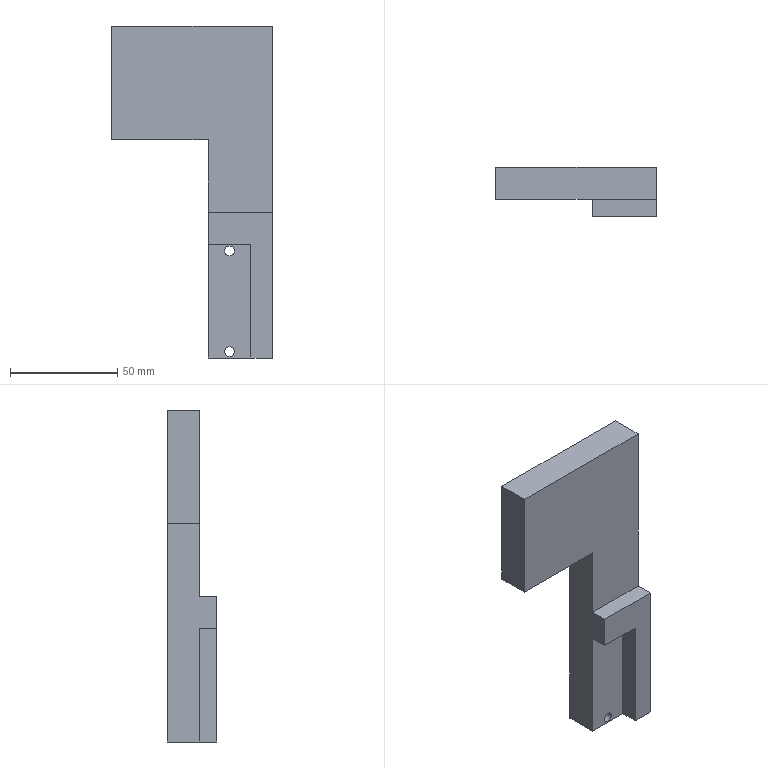Component | SolidWorks | TelescopicRodFixingBlock-1 | 1 solid | 24 faces | box 75 x 23 x 155 mm | volume 112588 mm3 | plane 15 | cylinder 9 | commonest cylinder face diameters 8 x5 4.5 x4
build123d program:
from build123d import *

# Parameters (mm, degrees)
BOSS_EXTRUDE1_DEPTH                             = 15
BOSS_EXTRUDE2_DEPTH                             = 8
M4_HEX_SOCKET_HEAD_CAP_SCREW_CBORE1_D           = 4.5
M4_HEX_SOCKET_HEAD_CAP_SCREW_CBORE1_CBORE_D     = 8
M4_HEX_SOCKET_HEAD_CAP_SCREW_CBORE1_CBORE_DEPTH = 4.6


with BuildPart() as part:
    # Sketch2 → Boss-Extrude1 (new body)
    with BuildSketch(Plane.XY):
        Polygon((10, 0.5), (-20, 0.5), (-20, 155.5), (55, 155.5), (55, 102.5), (10, 102.5), align=None)
    extrude(amount=BOSS_EXTRUDE1_DEPTH)

    # Sketch3 → Boss-Extrude2 (add)
    with BuildSketch(Plane(origin=(0, 0, 0), x_dir=(-1, 0, 0), z_dir=(0, 0, -1))):
        Polygon((20, 0.5), (10, 0.5), (10, 53.5), (-10, 53.5), (-10, 68.5), (20, 68.5), align=None)
    extrude(amount=BOSS_EXTRUDE2_DEPTH)

    # M4 Hex Socket Head Cap Screw CBORE1 (through all)
    with Locations(Plane.XY.offset(15)):
        with Locations((0, 50.5), (0, 3.5)):
            CounterBoreHole(M4_HEX_SOCKET_HEAD_CAP_SCREW_CBORE1_D / 2, M4_HEX_SOCKET_HEAD_CAP_SCREW_CBORE1_CBORE_D / 2, M4_HEX_SOCKET_HEAD_CAP_SCREW_CBORE1_CBORE_DEPTH)


solid = part.part

# Placed as in the assembly
solid = solid.moved(Location((-496.496, 273.496, 244.626), (-90, 0, 180)))
STEP:
#1=COLOUR_RGB('',0.7922,0.8196,0.9333);
#2=FILL_AREA_STYLE_COLOUR('',#1);
#3=FILL_AREA_STYLE('',(#2));
#4=SURFACE_STYLE_FILL_AREA(#3);
#5=SURFACE_SIDE_STYLE('',(#4));
#6=SURFACE_STYLE_USAGE(.BOTH.,#5);
#7=PRESENTATION_STYLE_ASSIGNMENT((#6));
#8=CARTESIAN_POINT('',(-19.39,11.177,11.619));
#9=VERTEX_POINT('',#8);
#10=CARTESIAN_POINT('',(-19.705,11.177,11.619));
#11=VERTEX_POINT('',#10);
#12=CARTESIAN_POINT('',(-19.547,11.177,11.619));
#13=DIRECTION('',(0.,1.,0.));
#14=DIRECTION('',(-1.,0.,0.));
#15=AXIS2_PLACEMENT_3D('',#12,#13,#14);
#16=CIRCLE('',#15,0.1575);
#17=EDGE_CURVE('',#9,#11,#16,.T.);
#18=ORIENTED_EDGE('',*,*,#17,.F.);
#19=CARTESIAN_POINT('',(-19.39,11.358,11.619));
#20=VERTEX_POINT('',#19);
#21=CARTESIAN_POINT('',(-19.39,11.358,11.619));
#22=DIRECTION('',(0.,1.,0.));
#23=VECTOR('',#22,39.37);
#24=LINE('',#21,#23);
#25=EDGE_CURVE('',#9,#20,#24,.T.);
#26=ORIENTED_EDGE('',*,*,#25,.T.);
#27=CARTESIAN_POINT('',(-19.705,11.358,11.619));
#28=VERTEX_POINT('',#27);
#29=CARTESIAN_POINT('',(-19.547,11.358,11.619));
#30=DIRECTION('',(0.,1.,0.));
#31=DIRECTION('',(-1.,0.,0.));
#32=AXIS2_PLACEMENT_3D('',#29,#30,#31);
#33=CIRCLE('',#32,0.1575);
#34=EDGE_CURVE('',#20,#28,#33,.T.);
#35=ORIENTED_EDGE('',*,*,#34,.T.);
#36=CARTESIAN_POINT('',(-19.705,11.358,11.619));
#37=DIRECTION('',(0.,1.,0.));
#38=VECTOR('',#37,39.37);
#39=LINE('',#36,#38);
#40=EDGE_CURVE('',#11,#28,#39,.T.);
#41=ORIENTED_EDGE('',*,*,#40,.F.);
#42=EDGE_LOOP('',(#18,#26,#35,#41));
#43=FACE_OUTER_BOUND('',#42,.T.);
#44=CARTESIAN_POINT('',(-19.547,11.358,11.619));
#45=DIRECTION('',(0.,1.,0.));
#46=DIRECTION('',(-1.,0.,0.));
#47=AXIS2_PLACEMENT_3D('',#44,#45,#46);
#48=CYLINDRICAL_SURFACE('',#47,0.1575);
#49=ADVANCED_FACE('',(#43),#48,.F.);
#50=CARTESIAN_POINT('',(-19.636,10.768,11.619));
#51=VERTEX_POINT('',#50);
#52=CARTESIAN_POINT('',(-19.459,10.768,11.619));
#53=VERTEX_POINT('',#52);
#54=CARTESIAN_POINT('',(-19.547,10.768,11.619));
#55=DIRECTION('',(-0.,-1.,-0.));
#56=DIRECTION('',(1.,0.,0.));
#57=AXIS2_PLACEMENT_3D('',#54,#55,#56);
#58=CIRCLE('',#57,0.08858);
#59=EDGE_CURVE('',#51,#53,#58,.T.);
#60=ORIENTED_EDGE('',*,*,#59,.T.);
#61=CARTESIAN_POINT('',(-19.459,11.177,11.619));
#62=VERTEX_POINT('',#61);
#63=CARTESIAN_POINT('',(-19.459,11.358,11.619));
#64=DIRECTION('',(0.,1.,0.));
#65=VECTOR('',#64,39.37);
#66=LINE('',#63,#65);
#67=EDGE_CURVE('',#53,#62,#66,.T.);
#68=ORIENTED_EDGE('',*,*,#67,.T.);
#69=CARTESIAN_POINT('',(-19.636,11.177,11.619));
#70=VERTEX_POINT('',#69);
#71=CARTESIAN_POINT('',(-19.547,11.177,11.619));
#72=DIRECTION('',(0.,1.,0.));
#73=DIRECTION('',(-1.,0.,0.));
#74=AXIS2_PLACEMENT_3D('',#71,#72,#73);
#75=CIRCLE('',#74,0.08858);
#76=EDGE_CURVE('',#62,#70,#75,.T.);
#77=ORIENTED_EDGE('',*,*,#76,.T.);
#78=CARTESIAN_POINT('',(-19.636,11.358,11.619));
#79=DIRECTION('',(0.,1.,0.));
#80=VECTOR('',#79,39.37);
#81=LINE('',#78,#80);
#82=EDGE_CURVE('',#51,#70,#81,.T.);
#83=ORIENTED_EDGE('',*,*,#82,.F.);
#84=EDGE_LOOP('',(#60,#68,#77,#83));
#85=FACE_OUTER_BOUND('',#84,.T.);
#86=CARTESIAN_POINT('',(-19.547,11.358,11.619));
#87=DIRECTION('',(0.,1.,0.));
#88=DIRECTION('',(-1.,0.,0.));
#89=AXIS2_PLACEMENT_3D('',#86,#87,#88);
#90=CYLINDRICAL_SURFACE('',#89,0.08858);
#91=ADVANCED_FACE('',(#85),#90,.F.);
#92=CARTESIAN_POINT('',(-19.636,10.768,9.769));
#93=VERTEX_POINT('',#92);
#94=CARTESIAN_POINT('',(-19.459,10.768,9.769));
#95=VERTEX_POINT('',#94);
#96=CARTESIAN_POINT('',(-19.547,10.768,9.769));
#97=DIRECTION('',(-0.,-1.,-0.));
#98=DIRECTION('',(1.,0.,0.));
#99=AXIS2_PLACEMENT_3D('',#96,#97,#98);
#100=CIRCLE('',#99,0.08858);
#101=EDGE_CURVE('',#93,#95,#100,.T.);
#102=ORIENTED_EDGE('',*,*,#101,.T.);
#103=CARTESIAN_POINT('',(-19.459,11.177,9.769));
#104=VERTEX_POINT('',#103);
#105=CARTESIAN_POINT('',(-19.459,11.358,9.769));
#106=DIRECTION('',(0.,1.,0.));
#107=VECTOR('',#106,39.37);
#108=LINE('',#105,#107);
#109=EDGE_CURVE('',#95,#104,#108,.T.);
#110=ORIENTED_EDGE('',*,*,#109,.T.);
#111=CARTESIAN_POINT('',(-19.636,11.177,9.769));
#112=VERTEX_POINT('',#111);
#113=CARTESIAN_POINT('',(-19.547,11.177,9.769));
#114=DIRECTION('',(0.,1.,0.));
#115=DIRECTION('',(-1.,0.,0.));
#116=AXIS2_PLACEMENT_3D('',#113,#114,#115);
#117=CIRCLE('',#116,0.08858);
#118=EDGE_CURVE('',#104,#112,#117,.T.);
#119=ORIENTED_EDGE('',*,*,#118,.T.);
#120=CARTESIAN_POINT('',(-19.636,11.358,9.769));
#121=DIRECTION('',(0.,1.,0.));
#122=VECTOR('',#121,39.37);
#123=LINE('',#120,#122);
#124=EDGE_CURVE('',#93,#112,#123,.T.);
#125=ORIENTED_EDGE('',*,*,#124,.F.);
#126=EDGE_LOOP('',(#102,#110,#119,#125));
#127=FACE_OUTER_BOUND('',#126,.T.);
#128=CARTESIAN_POINT('',(-19.547,11.358,9.769));
#129=DIRECTION('',(0.,1.,0.));
#130=DIRECTION('',(-1.,0.,0.));
#131=AXIS2_PLACEMENT_3D('',#128,#129,#130);
#132=CYLINDRICAL_SURFACE('',#131,0.08858);
#133=ADVANCED_FACE('',(#127),#132,.F.);
#134=CARTESIAN_POINT('',(-19.39,11.177,9.769));
#135=VERTEX_POINT('',#134);
#136=CARTESIAN_POINT('',(-19.443,11.177,9.651));
#137=VERTEX_POINT('',#136);
#138=CARTESIAN_POINT('',(-19.547,11.177,9.769));
#139=DIRECTION('',(0.,1.,0.));
#140=DIRECTION('',(-1.,0.,0.));
#141=AXIS2_PLACEMENT_3D('',#138,#139,#140);
#142=CIRCLE('',#141,0.1575);
#143=EDGE_CURVE('',#135,#137,#142,.T.);
#144=ORIENTED_EDGE('',*,*,#143,.F.);
#145=CARTESIAN_POINT('',(-19.39,11.358,9.769));
#146=VERTEX_POINT('',#145);
#147=CARTESIAN_POINT('',(-19.39,11.358,9.769));
#148=DIRECTION('',(0.,1.,0.));
#149=VECTOR('',#148,39.37);
#150=LINE('',#147,#149);
#151=EDGE_CURVE('',#135,#146,#150,.T.);
#152=ORIENTED_EDGE('',*,*,#151,.T.);
#153=CARTESIAN_POINT('',(-19.443,11.358,9.651));
#154=VERTEX_POINT('',#153);
#155=CARTESIAN_POINT('',(-19.547,11.358,9.769));
#156=DIRECTION('',(0.,1.,0.));
#157=DIRECTION('',(-1.,0.,0.));
#158=AXIS2_PLACEMENT_3D('',#155,#156,#157);
#159=CIRCLE('',#158,0.1575);
#160=EDGE_CURVE('',#146,#154,#159,.T.);
#161=ORIENTED_EDGE('',*,*,#160,.T.);
#162=CARTESIAN_POINT('',(-19.443,11.358,9.651));
#163=DIRECTION('',(0.,1.,0.));
#164=VECTOR('',#163,39.37);
#165=LINE('',#162,#164);
#166=EDGE_CURVE('',#137,#154,#165,.T.);
#167=ORIENTED_EDGE('',*,*,#166,.F.);
#168=EDGE_LOOP('',(#144,#152,#161,#167));
#169=FACE_OUTER_BOUND('',#168,.T.);
#170=CARTESIAN_POINT('',(-19.547,11.358,9.769));
#171=DIRECTION('',(0.,1.,0.));
#172=DIRECTION('',(-1.,0.,0.));
#173=AXIS2_PLACEMENT_3D('',#170,#171,#172);
#174=CYLINDRICAL_SURFACE('',#173,0.1575);
#175=ADVANCED_FACE('',(#169),#174,.F.);
#176=ORIENTED_EDGE('',*,*,#151,.F.);
#177=CARTESIAN_POINT('',(-19.705,11.177,9.769));
#178=VERTEX_POINT('',#177);
#179=CARTESIAN_POINT('',(-19.547,11.177,9.769));
#180=DIRECTION('',(0.,1.,0.));
#181=DIRECTION('',(-1.,0.,0.));
#182=AXIS2_PLACEMENT_3D('',#179,#180,#181);
#183=CIRCLE('',#182,0.1575);
#184=EDGE_CURVE('',#178,#135,#183,.T.);
#185=ORIENTED_EDGE('',*,*,#184,.F.);
#186=CARTESIAN_POINT('',(-19.705,11.358,9.769));
#187=VERTEX_POINT('',#186);
#188=CARTESIAN_POINT('',(-19.705,11.358,9.769));
#189=DIRECTION('',(0.,1.,0.));
#190=VECTOR('',#189,39.37);
#191=LINE('',#188,#190);
#192=EDGE_CURVE('',#178,#187,#191,.T.);
#193=ORIENTED_EDGE('',*,*,#192,.T.);
#194=CARTESIAN_POINT('',(-19.547,11.358,9.769));
#195=DIRECTION('',(0.,1.,0.));
#196=DIRECTION('',(-1.,0.,0.));
#197=AXIS2_PLACEMENT_3D('',#194,#195,#196);
#198=CIRCLE('',#197,0.1575);
#199=EDGE_CURVE('',#187,#146,#198,.T.);
#200=ORIENTED_EDGE('',*,*,#199,.T.);
#201=EDGE_LOOP('',(#176,#185,#193,#200));
#202=FACE_OUTER_BOUND('',#201,.T.);
#203=CARTESIAN_POINT('',(-19.547,11.358,9.769));
#204=DIRECTION('',(0.,1.,0.));
#205=DIRECTION('',(-1.,0.,0.));
#206=AXIS2_PLACEMENT_3D('',#203,#204,#205);
#207=CYLINDRICAL_SURFACE('',#206,0.1575);
#208=ADVANCED_FACE('',(#202),#207,.F.);
#209=CARTESIAN_POINT('',(-19.547,11.358,11.619));
#210=DIRECTION('',(0.,1.,0.));
#211=DIRECTION('',(-1.,0.,0.));
#212=AXIS2_PLACEMENT_3D('',#209,#210,#211);
#213=CIRCLE('',#212,0.1575);
#214=EDGE_CURVE('',#28,#20,#213,.T.);
#215=ORIENTED_EDGE('',*,*,#214,.F.);
#216=ORIENTED_EDGE('',*,*,#34,.F.);
#217=EDGE_LOOP('',(#215,#216));
#218=FACE_BOUND('',#217,.T.);
#219=CARTESIAN_POINT('',(-19.651,11.358,9.651));
#220=VERTEX_POINT('',#219);
#221=CARTESIAN_POINT('',(-19.547,11.358,9.769));
#222=DIRECTION('',(0.,1.,0.));
#223=DIRECTION('',(-1.,0.,0.));
#224=AXIS2_PLACEMENT_3D('',#221,#222,#223);
#225=CIRCLE('',#224,0.1575);
#226=EDGE_CURVE('',#220,#187,#225,.T.);
#227=ORIENTED_EDGE('',*,*,#226,.F.);
#228=CARTESIAN_POINT('',(-19.941,11.358,9.651));
#229=VERTEX_POINT('',#228);
#230=CARTESIAN_POINT('',(-19.941,11.358,9.651));
#231=DIRECTION('',(-1.,0.,-0.));
#232=VECTOR('',#231,39.37);
#233=LINE('',#230,#232);
#234=EDGE_CURVE('',#220,#229,#233,.T.);
#235=ORIENTED_EDGE('',*,*,#234,.T.);
#236=CARTESIAN_POINT('',(-19.941,11.358,13.666));
#237=VERTEX_POINT('',#236);
#238=CARTESIAN_POINT('',(-19.941,11.358,9.651));
#239=DIRECTION('',(-0.,-0.,1.));
#240=VECTOR('',#239,39.37);
#241=LINE('',#238,#240);
#242=EDGE_CURVE('',#229,#237,#241,.T.);
#243=ORIENTED_EDGE('',*,*,#242,.T.);
#244=CARTESIAN_POINT('',(-21.712,11.358,13.666));
#245=VERTEX_POINT('',#244);
#246=CARTESIAN_POINT('',(-19.941,11.358,13.666));
#247=DIRECTION('',(-1.,0.,-0.));
#248=VECTOR('',#247,39.37);
#249=LINE('',#246,#248);
#250=EDGE_CURVE('',#237,#245,#249,.T.);
#251=ORIENTED_EDGE('',*,*,#250,.T.);
#252=CARTESIAN_POINT('',(-21.712,11.358,15.753));
#253=VERTEX_POINT('',#252);
#254=CARTESIAN_POINT('',(-21.712,11.358,13.666));
#255=DIRECTION('',(-0.,-0.,1.));
#256=VECTOR('',#255,39.37);
#257=LINE('',#254,#256);
#258=EDGE_CURVE('',#245,#253,#257,.T.);
#259=ORIENTED_EDGE('',*,*,#258,.T.);
#260=CARTESIAN_POINT('',(-18.76,11.358,15.753));
#261=VERTEX_POINT('',#260);
#262=CARTESIAN_POINT('',(-18.76,11.358,15.753));
#263=DIRECTION('',(1.,-0.,0.));
#264=VECTOR('',#263,39.37);
#265=LINE('',#262,#264);
#266=EDGE_CURVE('',#253,#261,#265,.T.);
#267=ORIENTED_EDGE('',*,*,#266,.T.);
#268=CARTESIAN_POINT('',(-18.76,11.358,9.651));
#269=VERTEX_POINT('',#268);
#270=CARTESIAN_POINT('',(-18.76,11.358,9.651));
#271=DIRECTION('',(0.,0.,-1.));
#272=VECTOR('',#271,39.37);
#273=LINE('',#270,#272);
#274=EDGE_CURVE('',#261,#269,#273,.T.);
#275=ORIENTED_EDGE('',*,*,#274,.T.);
#276=CARTESIAN_POINT('',(-19.941,11.358,9.651));
#277=DIRECTION('',(-1.,0.,-0.));
#278=VECTOR('',#277,39.37);
#279=LINE('',#276,#278);
#280=EDGE_CURVE('',#269,#154,#279,.T.);
#281=ORIENTED_EDGE('',*,*,#280,.T.);
#282=ORIENTED_EDGE('',*,*,#160,.F.);
#283=ORIENTED_EDGE('',*,*,#199,.F.);
#284=EDGE_LOOP('',(#227,#235,#243,#251,#259,#267,#275,#281,#282,#283));
#285=FACE_OUTER_BOUND('',#284,.T.);
#286=CARTESIAN_POINT('',(-19.547,11.358,9.631));
#287=DIRECTION('',(-0.,-1.,-0.));
#288=DIRECTION('',(1.,-0.,0.));
#289=AXIS2_PLACEMENT_3D('',#286,#287,#288);
#290=PLANE('',#289);
#291=ADVANCED_FACE('',(#218,#285),#290,.F.);
#292=ORIENTED_EDGE('',*,*,#59,.F.);
#293=CARTESIAN_POINT('',(-19.547,10.768,11.619));
#294=DIRECTION('',(-0.,-1.,-0.));
#295=DIRECTION('',(1.,0.,0.));
#296=AXIS2_PLACEMENT_3D('',#293,#294,#295);
#297=CIRCLE('',#296,0.08858);
#298=EDGE_CURVE('',#53,#51,#297,.T.);
#299=ORIENTED_EDGE('',*,*,#298,.F.);
#300=EDGE_LOOP('',(#292,#299));
#301=FACE_BOUND('',#300,.T.);
#302=ORIENTED_EDGE('',*,*,#101,.F.);
#303=CARTESIAN_POINT('',(-19.547,10.768,9.769));
#304=DIRECTION('',(-0.,-1.,-0.));
#305=DIRECTION('',(1.,0.,0.));
#306=AXIS2_PLACEMENT_3D('',#303,#304,#305);
#307=CIRCLE('',#306,0.08858);
#308=EDGE_CURVE('',#95,#93,#307,.T.);
#309=ORIENTED_EDGE('',*,*,#308,.F.);
#310=EDGE_LOOP('',(#302,#309));
#311=FACE_BOUND('',#310,.T.);
#312=CARTESIAN_POINT('',(-19.153,10.768,11.737));
#313=VERTEX_POINT('',#312);
#314=CARTESIAN_POINT('',(-19.153,10.768,9.651));
#315=VERTEX_POINT('',#314);
#316=CARTESIAN_POINT('',(-19.153,10.768,9.651));
#317=DIRECTION('',(0.,0.,-1.));
#318=VECTOR('',#317,39.37);
#319=LINE('',#316,#318);
#320=EDGE_CURVE('',#313,#315,#319,.T.);
#321=ORIENTED_EDGE('',*,*,#320,.F.);
#322=CARTESIAN_POINT('',(-19.941,10.768,11.737));
#323=VERTEX_POINT('',#322);
#324=CARTESIAN_POINT('',(-19.941,10.768,11.737));
#325=DIRECTION('',(1.,-0.,0.));
#326=VECTOR('',#325,39.37);
#327=LINE('',#324,#326);
#328=EDGE_CURVE('',#323,#313,#327,.T.);
#329=ORIENTED_EDGE('',*,*,#328,.F.);
#330=CARTESIAN_POINT('',(-19.941,10.768,9.651));
#331=VERTEX_POINT('',#330);
#332=CARTESIAN_POINT('',(-19.941,10.768,9.651));
#333=DIRECTION('',(-0.,-0.,1.));
#334=VECTOR('',#333,39.37);
#335=LINE('',#332,#334);
#336=EDGE_CURVE('',#331,#323,#335,.T.);
#337=ORIENTED_EDGE('',*,*,#336,.F.);
#338=CARTESIAN_POINT('',(-19.941,10.768,9.651));
#339=DIRECTION('',(-1.,0.,-0.));
#340=VECTOR('',#339,39.37);
#341=LINE('',#338,#340);
#342=EDGE_CURVE('',#315,#331,#341,.T.);
#343=ORIENTED_EDGE('',*,*,#342,.F.);
#344=EDGE_LOOP('',(#321,#329,#337,#343));
#345=FACE_OUTER_BOUND('',#344,.T.);
#346=CARTESIAN_POINT('',(-19.547,10.768,9.631));
#347=DIRECTION('',(-0.,-1.,-0.));
#348=DIRECTION('',(1.,-0.,0.));
#349=AXIS2_PLACEMENT_3D('',#346,#347,#348);
#350=PLANE('',#349);
#351=ADVANCED_FACE('',(#301,#311,#345),#350,.T.);
#352=ORIENTED_EDGE('',*,*,#336,.T.);
#353=CARTESIAN_POINT('',(-19.941,10.453,11.737));
#354=VERTEX_POINT('',#353);
#355=CARTESIAN_POINT('',(-19.941,10.453,11.737));
#356=DIRECTION('',(0.,1.,0.));
#357=VECTOR('',#356,39.37);
#358=LINE('',#355,#357);
#359=EDGE_CURVE('',#354,#323,#358,.T.);
#360=ORIENTED_EDGE('',*,*,#359,.F.);
#361=CARTESIAN_POINT('',(-19.941,10.453,12.328));
#362=VERTEX_POINT('',#361);
#363=CARTESIAN_POINT('',(-19.941,10.453,11.737));
#364=DIRECTION('',(0.,0.,-1.));
#365=VECTOR('',#364,39.37);
#366=LINE('',#363,#365);
#367=EDGE_CURVE('',#362,#354,#366,.T.);
#368=ORIENTED_EDGE('',*,*,#367,.F.);
#369=CARTESIAN_POINT('',(-19.941,10.768,12.328));
#370=VERTEX_POINT('',#369);
#371=CARTESIAN_POINT('',(-19.941,10.453,12.328));
#372=DIRECTION('',(0.,1.,0.));
#373=VECTOR('',#372,39.37);
#374=LINE('',#371,#373);
#375=EDGE_CURVE('',#362,#370,#374,.T.);
#376=ORIENTED_EDGE('',*,*,#375,.T.);
#377=CARTESIAN_POINT('',(-19.941,10.768,13.666));
#378=VERTEX_POINT('',#377);
#379=CARTESIAN_POINT('',(-19.941,10.768,9.651));
#380=DIRECTION('',(-0.,-0.,1.));
#381=VECTOR('',#380,39.37);
#382=LINE('',#379,#381);
#383=EDGE_CURVE('',#370,#378,#382,.T.);
#384=ORIENTED_EDGE('',*,*,#383,.T.);
#385=CARTESIAN_POINT('',(-19.941,11.358,13.666));
#386=DIRECTION('',(-0.,-1.,-0.));
#387=VECTOR('',#386,39.37);
#388=LINE('',#385,#387);
#389=EDGE_CURVE('',#237,#378,#388,.T.);
#390=ORIENTED_EDGE('',*,*,#389,.F.);
#391=ORIENTED_EDGE('',*,*,#242,.F.);
#392=CARTESIAN_POINT('',(-19.941,11.358,9.651));
#393=DIRECTION('',(-0.,-1.,-0.));
#394=VECTOR('',#393,39.37);
#395=LINE('',#392,#394);
#396=EDGE_CURVE('',#229,#331,#395,.T.);
#397=ORIENTED_EDGE('',*,*,#396,.T.);
#398=EDGE_LOOP('',(#352,#360,#368,#376,#384,#390,#391,#397));
#399=FACE_OUTER_BOUND('',#398,.T.);
#400=CARTESIAN_POINT('',(-19.941,11.358,9.651));
#401=DIRECTION('',(1.,-0.,0.));
#402=DIRECTION('',(0.,1.,0.));
#403=AXIS2_PLACEMENT_3D('',#400,#401,#402);
#404=PLANE('',#403);
#405=ADVANCED_FACE('',(#399),#404,.F.);
#406=CARTESIAN_POINT('',(-21.712,10.768,13.666));
#407=VERTEX_POINT('',#406);
#408=CARTESIAN_POINT('',(-19.941,10.768,13.666));
#409=DIRECTION('',(-1.,0.,-0.));
#410=VECTOR('',#409,39.37);
#411=LINE('',#408,#410);
#412=EDGE_CURVE('',#378,#407,#411,.T.);
#413=ORIENTED_EDGE('',*,*,#412,.T.);
#414=CARTESIAN_POINT('',(-21.712,11.358,13.666));
#415=DIRECTION('',(-0.,-1.,-0.));
#416=VECTOR('',#415,39.37);
#417=LINE('',#414,#416);
#418=EDGE_CURVE('',#245,#407,#417,.T.);
#419=ORIENTED_EDGE('',*,*,#418,.F.);
#420=ORIENTED_EDGE('',*,*,#250,.F.);
#421=ORIENTED_EDGE('',*,*,#389,.T.);
#422=EDGE_LOOP('',(#413,#419,#420,#421));
#423=FACE_OUTER_BOUND('',#422,.T.);
#424=CARTESIAN_POINT('',(-19.941,11.358,13.666));
#425=DIRECTION('',(-0.,-0.,1.));
#426=DIRECTION('',(0.,1.,0.));
#427=AXIS2_PLACEMENT_3D('',#424,#425,#426);
#428=PLANE('',#427);
#429=ADVANCED_FACE('',(#423),#428,.F.);
#430=CARTESIAN_POINT('',(-21.712,10.768,15.753));
#431=VERTEX_POINT('',#430);
#432=CARTESIAN_POINT('',(-21.712,10.768,13.666));
#433=DIRECTION('',(-0.,-0.,1.));
#434=VECTOR('',#433,39.37);
#435=LINE('',#432,#434);
#436=EDGE_CURVE('',#407,#431,#435,.T.);
#437=ORIENTED_EDGE('',*,*,#436,.T.);
#438=CARTESIAN_POINT('',(-21.712,11.358,15.753));
#439=DIRECTION('',(-0.,-1.,-0.));
#440=VECTOR('',#439,39.37);
#441=LINE('',#438,#440);
#442=EDGE_CURVE('',#253,#431,#441,.T.);
#443=ORIENTED_EDGE('',*,*,#442,.F.);
#444=ORIENTED_EDGE('',*,*,#258,.F.);
#445=ORIENTED_EDGE('',*,*,#418,.T.);
#446=EDGE_LOOP('',(#437,#443,#444,#445));
#447=FACE_OUTER_BOUND('',#446,.T.);
#448=CARTESIAN_POINT('',(-21.712,11.358,13.666));
#449=DIRECTION('',(1.,-0.,0.));
#450=DIRECTION('',(0.,1.,0.));
#451=AXIS2_PLACEMENT_3D('',#448,#449,#450);
#452=PLANE('',#451);
#453=ADVANCED_FACE('',(#447),#452,.F.);
#454=CARTESIAN_POINT('',(-18.76,10.768,15.753));
#455=VERTEX_POINT('',#454);
#456=CARTESIAN_POINT('',(-18.76,10.768,15.753));
#457=DIRECTION('',(1.,-0.,0.));
#458=VECTOR('',#457,39.37);
#459=LINE('',#456,#458);
#460=EDGE_CURVE('',#431,#455,#459,.T.);
#461=ORIENTED_EDGE('',*,*,#460,.T.);
#462=CARTESIAN_POINT('',(-18.76,11.358,15.753));
#463=DIRECTION('',(-0.,-1.,-0.));
#464=VECTOR('',#463,39.37);
#465=LINE('',#462,#464);
#466=EDGE_CURVE('',#261,#455,#465,.T.);
#467=ORIENTED_EDGE('',*,*,#466,.F.);
#468=ORIENTED_EDGE('',*,*,#266,.F.);
#469=ORIENTED_EDGE('',*,*,#442,.T.);
#470=EDGE_LOOP('',(#461,#467,#468,#469));
#471=FACE_OUTER_BOUND('',#470,.T.);
#472=CARTESIAN_POINT('',(-18.76,11.358,15.753));
#473=DIRECTION('',(0.,0.,-1.));
#474=DIRECTION('',(-0.,-1.,-0.));
#475=AXIS2_PLACEMENT_3D('',#472,#473,#474);
#476=PLANE('',#475);
#477=ADVANCED_FACE('',(#471),#476,.F.);
#478=CARTESIAN_POINT('',(-18.76,10.768,12.328));
#479=VERTEX_POINT('',#478);
#480=CARTESIAN_POINT('',(-18.76,10.768,9.651));
#481=DIRECTION('',(0.,0.,-1.));
#482=VECTOR('',#481,39.37);
#483=LINE('',#480,#482);
#484=EDGE_CURVE('',#455,#479,#483,.T.);
#485=ORIENTED_EDGE('',*,*,#484,.T.);
#486=CARTESIAN_POINT('',(-18.76,10.453,12.328));
#487=VERTEX_POINT('',#486);
#488=CARTESIAN_POINT('',(-18.76,10.453,12.328));
#489=DIRECTION('',(0.,1.,0.));
#490=VECTOR('',#489,39.37);
#491=LINE('',#488,#490);
#492=EDGE_CURVE('',#487,#479,#491,.T.);
#493=ORIENTED_EDGE('',*,*,#492,.F.);
#494=CARTESIAN_POINT('',(-18.76,10.453,9.651));
#495=VERTEX_POINT('',#494);
#496=CARTESIAN_POINT('',(-18.76,10.453,9.651));
#497=DIRECTION('',(-0.,-0.,1.));
#498=VECTOR('',#497,39.37);
#499=LINE('',#496,#498);
#500=EDGE_CURVE('',#495,#487,#499,.T.);
#501=ORIENTED_EDGE('',*,*,#500,.F.);
#502=CARTESIAN_POINT('',(-18.76,11.358,9.651));
#503=DIRECTION('',(-0.,-1.,-0.));
#504=VECTOR('',#503,39.37);
#505=LINE('',#502,#504);
#506=EDGE_CURVE('',#269,#495,#505,.T.);
#507=ORIENTED_EDGE('',*,*,#506,.F.);
#508=ORIENTED_EDGE('',*,*,#274,.F.);
#509=ORIENTED_EDGE('',*,*,#466,.T.);
#510=EDGE_LOOP('',(#485,#493,#501,#507,#508,#509));
#511=FACE_OUTER_BOUND('',#510,.T.);
#512=CARTESIAN_POINT('',(-18.76,11.358,9.651));
#513=DIRECTION('',(-1.,0.,-0.));
#514=DIRECTION('',(-0.,-1.,-0.));
#515=AXIS2_PLACEMENT_3D('',#512,#513,#514);
#516=PLANE('',#515);
#517=ADVANCED_FACE('',(#511),#516,.F.);
#518=CARTESIAN_POINT('',(-19.651,11.177,9.651));
#519=VERTEX_POINT('',#518);
#520=CARTESIAN_POINT('',(-19.941,11.177,9.651));
#521=DIRECTION('',(1.,-0.,0.));
#522=VECTOR('',#521,39.37);
#523=LINE('',#520,#522);
#524=EDGE_CURVE('',#519,#137,#523,.T.);
#525=ORIENTED_EDGE('',*,*,#524,.T.);
#526=ORIENTED_EDGE('',*,*,#166,.T.);
#527=ORIENTED_EDGE('',*,*,#280,.F.);
#528=ORIENTED_EDGE('',*,*,#506,.T.);
#529=CARTESIAN_POINT('',(-19.153,10.453,9.651));
#530=VERTEX_POINT('',#529);
#531=CARTESIAN_POINT('',(-18.76,10.453,9.651));
#532=DIRECTION('',(1.,-0.,0.));
#533=VECTOR('',#532,39.37);
#534=LINE('',#531,#533);
#535=EDGE_CURVE('',#530,#495,#534,.T.);
#536=ORIENTED_EDGE('',*,*,#535,.F.);
#537=CARTESIAN_POINT('',(-19.153,10.453,9.651));
#538=DIRECTION('',(0.,1.,0.));
#539=VECTOR('',#538,39.37);
#540=LINE('',#537,#539);
#541=EDGE_CURVE('',#530,#315,#540,.T.);
#542=ORIENTED_EDGE('',*,*,#541,.T.);
#543=ORIENTED_EDGE('',*,*,#342,.T.);
#544=ORIENTED_EDGE('',*,*,#396,.F.);
#545=ORIENTED_EDGE('',*,*,#234,.F.);
#546=CARTESIAN_POINT('',(-19.651,11.358,9.651));
#547=DIRECTION('',(-0.,-1.,-0.));
#548=VECTOR('',#547,39.37);
#549=LINE('',#546,#548);
#550=EDGE_CURVE('',#220,#519,#549,.T.);
#551=ORIENTED_EDGE('',*,*,#550,.T.);
#552=EDGE_LOOP('',(#525,#526,#527,#528,#536,#542,#543,#544,#545,#551));
#553=FACE_OUTER_BOUND('',#552,.T.);
#554=CARTESIAN_POINT('',(-19.941,11.358,9.651));
#555=DIRECTION('',(-0.,-0.,1.));
#556=DIRECTION('',(1.,-0.,0.));
#557=AXIS2_PLACEMENT_3D('',#554,#555,#556);
#558=PLANE('',#557);
#559=ADVANCED_FACE('',(#553),#558,.F.);
#560=CARTESIAN_POINT('',(-19.941,10.768,12.328));
#561=DIRECTION('',(-1.,0.,-0.));
#562=VECTOR('',#561,39.37);
#563=LINE('',#560,#562);
#564=EDGE_CURVE('',#479,#370,#563,.T.);
#565=ORIENTED_EDGE('',*,*,#564,.F.);
#566=ORIENTED_EDGE('',*,*,#484,.F.);
#567=ORIENTED_EDGE('',*,*,#460,.F.);
#568=ORIENTED_EDGE('',*,*,#436,.F.);
#569=ORIENTED_EDGE('',*,*,#412,.F.);
#570=ORIENTED_EDGE('',*,*,#383,.F.);
#571=EDGE_LOOP('',(#565,#566,#567,#568,#569,#570));
#572=FACE_OUTER_BOUND('',#571,.T.);
#573=CARTESIAN_POINT('',(-19.547,10.768,9.631));
#574=DIRECTION('',(-0.,-1.,-0.));
#575=DIRECTION('',(1.,-0.,0.));
#576=AXIS2_PLACEMENT_3D('',#573,#574,#575);
#577=PLANE('',#576);
#578=ADVANCED_FACE('',(#572),#577,.T.);
#579=ORIENTED_EDGE('',*,*,#564,.T.);
#580=ORIENTED_EDGE('',*,*,#375,.F.);
#581=CARTESIAN_POINT('',(-19.941,10.453,12.328));
#582=DIRECTION('',(-1.,0.,-0.));
#583=VECTOR('',#582,39.37);
#584=LINE('',#581,#583);
#585=EDGE_CURVE('',#487,#362,#584,.T.);
#586=ORIENTED_EDGE('',*,*,#585,.F.);
#587=ORIENTED_EDGE('',*,*,#492,.T.);
#588=EDGE_LOOP('',(#579,#580,#586,#587));
#589=FACE_OUTER_BOUND('',#588,.T.);
#590=CARTESIAN_POINT('',(-19.941,10.453,12.328));
#591=DIRECTION('',(0.,0.,-1.));
#592=DIRECTION('',(-0.,-1.,-0.));
#593=AXIS2_PLACEMENT_3D('',#590,#591,#592);
#594=PLANE('',#593);
#595=ADVANCED_FACE('',(#589),#594,.F.);
#596=ORIENTED_EDGE('',*,*,#328,.T.);
#597=CARTESIAN_POINT('',(-19.153,10.453,11.737));
#598=VERTEX_POINT('',#597);
#599=CARTESIAN_POINT('',(-19.153,10.453,11.737));
#600=DIRECTION('',(0.,1.,0.));
#601=VECTOR('',#600,39.37);
#602=LINE('',#599,#601);
#603=EDGE_CURVE('',#598,#313,#602,.T.);
#604=ORIENTED_EDGE('',*,*,#603,.F.);
#605=CARTESIAN_POINT('',(-19.941,10.453,11.737));
#606=DIRECTION('',(1.,-0.,0.));
#607=VECTOR('',#606,39.37);
#608=LINE('',#605,#607);
#609=EDGE_CURVE('',#354,#598,#608,.T.);
#610=ORIENTED_EDGE('',*,*,#609,.F.);
#611=ORIENTED_EDGE('',*,*,#359,.T.);
#612=EDGE_LOOP('',(#596,#604,#610,#611));
#613=FACE_OUTER_BOUND('',#612,.T.);
#614=CARTESIAN_POINT('',(-19.941,10.453,11.737));
#615=DIRECTION('',(-0.,-0.,1.));
#616=DIRECTION('',(0.,1.,0.));
#617=AXIS2_PLACEMENT_3D('',#614,#615,#616);
#618=PLANE('',#617);
#619=ADVANCED_FACE('',(#613),#618,.F.);
#620=ORIENTED_EDGE('',*,*,#320,.T.);
#621=ORIENTED_EDGE('',*,*,#541,.F.);
#622=CARTESIAN_POINT('',(-19.153,10.453,9.651));
#623=DIRECTION('',(0.,0.,-1.));
#624=VECTOR('',#623,39.37);
#625=LINE('',#622,#624);
#626=EDGE_CURVE('',#598,#530,#625,.T.);
#627=ORIENTED_EDGE('',*,*,#626,.F.);
#628=ORIENTED_EDGE('',*,*,#603,.T.);
#629=EDGE_LOOP('',(#620,#621,#627,#628));
#630=FACE_OUTER_BOUND('',#629,.T.);
#631=CARTESIAN_POINT('',(-19.153,10.453,9.651));
#632=DIRECTION('',(1.,-0.,0.));
#633=DIRECTION('',(0.,0.,-1.));
#634=AXIS2_PLACEMENT_3D('',#631,#632,#633);
#635=PLANE('',#634);
#636=ADVANCED_FACE('',(#630),#635,.F.);
#637=ORIENTED_EDGE('',*,*,#500,.T.);
#638=ORIENTED_EDGE('',*,*,#585,.T.);
#639=ORIENTED_EDGE('',*,*,#367,.T.);
#640=ORIENTED_EDGE('',*,*,#609,.T.);
#641=ORIENTED_EDGE('',*,*,#626,.T.);
#642=ORIENTED_EDGE('',*,*,#535,.T.);
#643=EDGE_LOOP('',(#637,#638,#639,#640,#641,#642));
#644=FACE_OUTER_BOUND('',#643,.T.);
#645=CARTESIAN_POINT('',(-19.547,10.453,9.631));
#646=DIRECTION('',(0.,1.,0.));
#647=DIRECTION('',(-1.,0.,-0.));
#648=AXIS2_PLACEMENT_3D('',#645,#646,#647);
#649=PLANE('',#648);
#650=ADVANCED_FACE('',(#644),#649,.F.);
#651=CARTESIAN_POINT('',(-19.547,11.177,9.769));
#652=DIRECTION('',(0.,1.,0.));
#653=DIRECTION('',(-1.,0.,0.));
#654=AXIS2_PLACEMENT_3D('',#651,#652,#653);
#655=CIRCLE('',#654,0.08858);
#656=EDGE_CURVE('',#112,#104,#655,.T.);
#657=ORIENTED_EDGE('',*,*,#656,.F.);
#658=ORIENTED_EDGE('',*,*,#118,.F.);
#659=EDGE_LOOP('',(#657,#658));
#660=FACE_BOUND('',#659,.T.);
#661=CARTESIAN_POINT('',(-19.547,11.177,9.769));
#662=DIRECTION('',(0.,1.,0.));
#663=DIRECTION('',(-1.,0.,0.));
#664=AXIS2_PLACEMENT_3D('',#661,#662,#663);
#665=CIRCLE('',#664,0.1575);
#666=EDGE_CURVE('',#519,#178,#665,.T.);
#667=ORIENTED_EDGE('',*,*,#666,.T.);
#668=ORIENTED_EDGE('',*,*,#184,.T.);
#669=ORIENTED_EDGE('',*,*,#143,.T.);
#670=ORIENTED_EDGE('',*,*,#524,.F.);
#671=EDGE_LOOP('',(#667,#668,#669,#670));
#672=FACE_OUTER_BOUND('',#671,.T.);
#673=CARTESIAN_POINT('',(-19.636,11.177,9.769));
#674=DIRECTION('',(-0.,-1.,-0.));
#675=DIRECTION('',(1.,-0.,0.));
#676=AXIS2_PLACEMENT_3D('',#673,#674,#675);
#677=PLANE('',#676);
#678=ADVANCED_FACE('',(#660,#672),#677,.F.);
#679=ORIENTED_EDGE('',*,*,#192,.F.);
#680=ORIENTED_EDGE('',*,*,#666,.F.);
#681=ORIENTED_EDGE('',*,*,#550,.F.);
#682=ORIENTED_EDGE('',*,*,#226,.T.);
#683=EDGE_LOOP('',(#679,#680,#681,#682));
#684=FACE_OUTER_BOUND('',#683,.T.);
#685=CARTESIAN_POINT('',(-19.547,11.358,9.769));
#686=DIRECTION('',(0.,1.,0.));
#687=DIRECTION('',(-1.,0.,0.));
#688=AXIS2_PLACEMENT_3D('',#685,#686,#687);
#689=CYLINDRICAL_SURFACE('',#688,0.1575);
#690=ADVANCED_FACE('',(#684),#689,.F.);
#691=ORIENTED_EDGE('',*,*,#109,.F.);
#692=ORIENTED_EDGE('',*,*,#308,.T.);
#693=ORIENTED_EDGE('',*,*,#124,.T.);
#694=ORIENTED_EDGE('',*,*,#656,.T.);
#695=EDGE_LOOP('',(#691,#692,#693,#694));
#696=FACE_OUTER_BOUND('',#695,.T.);
#697=CARTESIAN_POINT('',(-19.547,11.358,9.769));
#698=DIRECTION('',(0.,1.,0.));
#699=DIRECTION('',(-1.,0.,0.));
#700=AXIS2_PLACEMENT_3D('',#697,#698,#699);
#701=CYLINDRICAL_SURFACE('',#700,0.08858);
#702=ADVANCED_FACE('',(#696),#701,.F.);
#703=ORIENTED_EDGE('',*,*,#67,.F.);
#704=ORIENTED_EDGE('',*,*,#298,.T.);
#705=ORIENTED_EDGE('',*,*,#82,.T.);
#706=CARTESIAN_POINT('',(-19.547,11.177,11.619));
#707=DIRECTION('',(0.,1.,0.));
#708=DIRECTION('',(-1.,0.,0.));
#709=AXIS2_PLACEMENT_3D('',#706,#707,#708);
#710=CIRCLE('',#709,0.08858);
#711=EDGE_CURVE('',#70,#62,#710,.T.);
#712=ORIENTED_EDGE('',*,*,#711,.T.);
#713=EDGE_LOOP('',(#703,#704,#705,#712));
#714=FACE_OUTER_BOUND('',#713,.T.);
#715=CARTESIAN_POINT('',(-19.547,11.358,11.619));
#716=DIRECTION('',(0.,1.,0.));
#717=DIRECTION('',(-1.,0.,0.));
#718=AXIS2_PLACEMENT_3D('',#715,#716,#717);
#719=CYLINDRICAL_SURFACE('',#718,0.08858);
#720=ADVANCED_FACE('',(#714),#719,.F.);
#721=ORIENTED_EDGE('',*,*,#711,.F.);
#722=ORIENTED_EDGE('',*,*,#76,.F.);
#723=EDGE_LOOP('',(#721,#722));
#724=FACE_BOUND('',#723,.T.);
#725=CARTESIAN_POINT('',(-19.547,11.177,11.619));
#726=DIRECTION('',(0.,1.,0.));
#727=DIRECTION('',(-1.,0.,0.));
#728=AXIS2_PLACEMENT_3D('',#725,#726,#727);
#729=CIRCLE('',#728,0.1575);
#730=EDGE_CURVE('',#11,#9,#729,.T.);
#731=ORIENTED_EDGE('',*,*,#730,.T.);
#732=ORIENTED_EDGE('',*,*,#17,.T.);
#733=EDGE_LOOP('',(#731,#732));
#734=FACE_OUTER_BOUND('',#733,.T.);
#735=CARTESIAN_POINT('',(-19.636,11.177,11.619));
#736=DIRECTION('',(-0.,-1.,-0.));
#737=DIRECTION('',(1.,-0.,0.));
#738=AXIS2_PLACEMENT_3D('',#735,#736,#737);
#739=PLANE('',#738);
#740=ADVANCED_FACE('',(#724,#734),#739,.F.);
#741=ORIENTED_EDGE('',*,*,#25,.F.);
#742=ORIENTED_EDGE('',*,*,#730,.F.);
#743=ORIENTED_EDGE('',*,*,#40,.T.);
#744=ORIENTED_EDGE('',*,*,#214,.T.);
#745=EDGE_LOOP('',(#741,#742,#743,#744));
#746=FACE_OUTER_BOUND('',#745,.T.);
#747=CARTESIAN_POINT('',(-19.547,11.358,11.619));
#748=DIRECTION('',(0.,1.,0.));
#749=DIRECTION('',(-1.,0.,0.));
#750=AXIS2_PLACEMENT_3D('',#747,#748,#749);
#751=CYLINDRICAL_SURFACE('',#750,0.1575);
#752=ADVANCED_FACE('',(#746),#751,.F.);
#753=CLOSED_SHELL('',(#49,#91,#133,#175,#208,#291,#351,#405,#429,#453,#477,#517,#559,#578,#595,#619,#636,#650,#678,#690,#702,#720,#740,#752));
#754=MANIFOLD_SOLID_BREP('',#753);
#755=STYLED_ITEM('',(#7),#754);
#756=PRESENTATION_LAYER_ASSIGNMENT('','',(#755));
#757=CARTESIAN_POINT('',(0.,0.,0.));
#758=DIRECTION('',(0.,0.,1.));
#759=DIRECTION('',(1.,0.,0.));
#760=AXIS2_PLACEMENT_3D('',#757,#758,#759);
#761=(LENGTH_UNIT()NAMED_UNIT(*)SI_UNIT($,.METRE.));
#762=LENGTH_MEASURE_WITH_UNIT(LENGTH_MEASURE(0.0254),#761);
#763=DIMENSIONAL_EXPONENTS(1.,0.,0.,0.,0.,0.,0.);
#764=(CONVERSION_BASED_UNIT('',#762)LENGTH_UNIT()NAMED_UNIT(#763));
#765=UNCERTAINTY_MEASURE_WITH_UNIT(LENGTH_MEASURE(0.00001),#764,'','');
#766=(NAMED_UNIT(*)PLANE_ANGLE_UNIT()SI_UNIT($,.RADIAN.));
#767=(NAMED_UNIT(*)SI_UNIT($,.STERADIAN.)SOLID_ANGLE_UNIT());
#768=(GEOMETRIC_REPRESENTATION_CONTEXT(3)GLOBAL_UNCERTAINTY_ASSIGNED_CONTEXT((#765))GLOBAL_UNIT_ASSIGNED_CONTEXT((#764,#766,#767))REPRESENTATION_CONTEXT('',''));
#769=ADVANCED_BREP_SHAPE_REPRESENTATION('',(#754,#760),#768);
#770=(LENGTH_UNIT()NAMED_UNIT(*)SI_UNIT($,.METRE.));
#771=LENGTH_MEASURE_WITH_UNIT(LENGTH_MEASURE(0.0254),#770);
#772=DIMENSIONAL_EXPONENTS(1.,0.,0.,0.,0.,0.,0.);
#773=(CONVERSION_BASED_UNIT('',#771)LENGTH_UNIT()NAMED_UNIT(#772));
#774=UNCERTAINTY_MEASURE_WITH_UNIT(LENGTH_MEASURE(0.00001),#773,'','');
#775=(NAMED_UNIT(*)PLANE_ANGLE_UNIT()SI_UNIT($,.RADIAN.));
#776=(NAMED_UNIT(*)SI_UNIT($,.STERADIAN.)SOLID_ANGLE_UNIT());
#777=(GEOMETRIC_REPRESENTATION_CONTEXT(3)GLOBAL_UNCERTAINTY_ASSIGNED_CONTEXT((#774))GLOBAL_UNIT_ASSIGNED_CONTEXT((#773,#775,#776))REPRESENTATION_CONTEXT('',''));
#778=MECHANICAL_DESIGN_GEOMETRIC_PRESENTATION_REPRESENTATION('',(#755),#777);